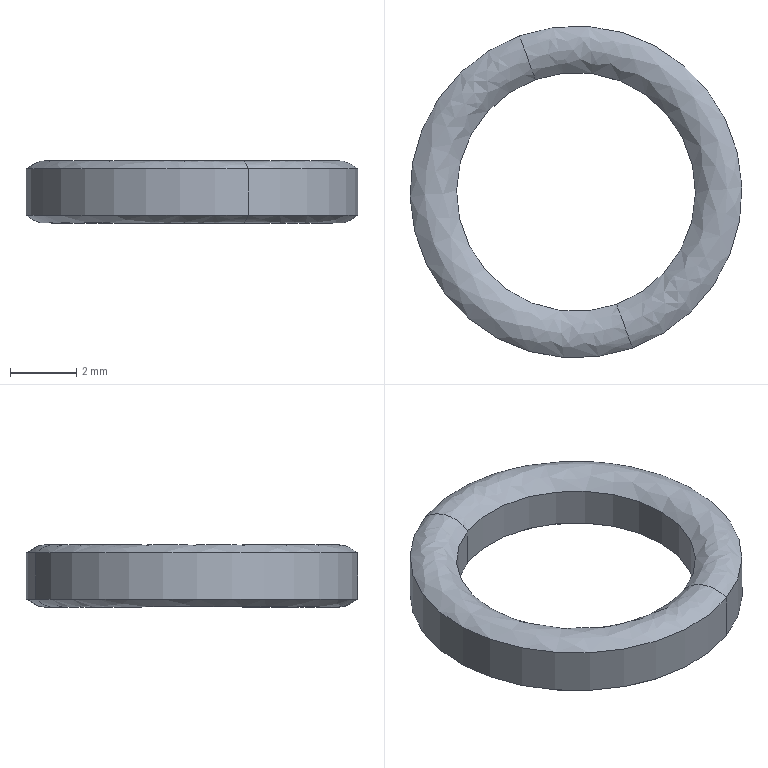Component | SolidWorks | NPB7-3 | 1 solid | 8 faces | box 10 x 10 x 1.9 mm | volume 65 mm3 | spline 4 | cylinder 4 | commonest cylinder face diameters 7.2 x2 10 x2
STEP:
#1=COLOUR_RGB('',0.7922,0.8196,0.9333);
#2=FILL_AREA_STYLE_COLOUR('',#1);
#3=FILL_AREA_STYLE('',(#2));
#4=SURFACE_STYLE_FILL_AREA(#3);
#5=SURFACE_SIDE_STYLE('',(#4));
#6=SURFACE_STYLE_USAGE(.BOTH.,#5);
#7=PRESENTATION_STYLE_ASSIGNMENT((#6));
#8=CARTESIAN_POINT('',(-0.06694,-1.587,0.3009));
#9=VERTEX_POINT('',#8);
#10=CARTESIAN_POINT('',(0.06694,-1.957,0.3009));
#11=VERTEX_POINT('',#10);
#12=CARTESIAN_POINT('',(0.,-1.772,0.3009));
#13=DIRECTION('',(-0.,-0.,1.));
#14=DIRECTION('',(-0.34,0.9404,0.));
#15=AXIS2_PLACEMENT_3D('',#12,#13,#14);
#16=CIRCLE('',#15,0.1969);
#17=EDGE_CURVE('',#9,#11,#16,.T.);
#18=ORIENTED_EDGE('',*,*,#17,.T.);
#19=CARTESIAN_POINT('',(0.04819,-1.905,0.2966));
#20=VERTEX_POINT('',#19);
#21=CARTESIAN_POINT('',(0.05823,-1.933,0.2736));
#22=DIRECTION('',(-0.9404,-0.34,-0.));
#23=DIRECTION('',(0.34,-0.9404,0.));
#24=AXIS2_PLACEMENT_3D('',#21,#22,#23);
#25=CIRCLE('',#24,0.0374);
#26=EDGE_CURVE('',#11,#20,#25,.T.);
#27=ORIENTED_EDGE('',*,*,#26,.T.);
#28=CARTESIAN_POINT('',(-0.04819,-1.638,0.2966));
#29=VERTEX_POINT('',#28);
#30=CARTESIAN_POINT('',(0.,-1.772,0.2966));
#31=DIRECTION('',(-0.,-0.,1.));
#32=DIRECTION('',(-0.34,0.9404,0.));
#33=AXIS2_PLACEMENT_3D('',#30,#31,#32);
#34=CIRCLE('',#33,0.1417);
#35=EDGE_CURVE('',#29,#20,#34,.T.);
#36=ORIENTED_EDGE('',*,*,#35,.F.);
#37=CARTESIAN_POINT('',(-0.05823,-1.611,0.2736));
#38=DIRECTION('',(0.9404,0.34,0.));
#39=DIRECTION('',(-0.34,0.9404,0.));
#40=AXIS2_PLACEMENT_3D('',#37,#38,#39);
#41=CIRCLE('',#40,0.0374);
#42=EDGE_CURVE('',#9,#29,#41,.T.);
#43=ORIENTED_EDGE('',*,*,#42,.F.);
#44=EDGE_LOOP('',(#18,#27,#36,#43));
#45=FACE_OUTER_BOUND('',#44,.T.);
#46=CARTESIAN_POINT('',(0.06694,-1.957,0.3009));
#47=CARTESIAN_POINT('',(-0.3033,-2.091,0.3009));
#48=CARTESIAN_POINT('',(-0.4372,-1.72,0.3009));
#49=CARTESIAN_POINT('',(-0.06694,-1.587,0.3009));
#50=CARTESIAN_POINT('',(0.06109,-1.941,0.317));
#51=CARTESIAN_POINT('',(-0.2768,-2.063,0.317));
#52=CARTESIAN_POINT('',(-0.399,-1.725,0.317));
#53=CARTESIAN_POINT('',(-0.06109,-1.603,0.317));
#54=CARTESIAN_POINT('',(0.05311,-1.919,0.3152));
#55=CARTESIAN_POINT('',(-0.2407,-2.025,0.3152));
#56=CARTESIAN_POINT('',(-0.3469,-1.731,0.3152));
#57=CARTESIAN_POINT('',(-0.05311,-1.625,0.3152));
#58=CARTESIAN_POINT('',(0.04819,-1.905,0.2966));
#59=CARTESIAN_POINT('',(-0.2184,-2.001,0.2966));
#60=CARTESIAN_POINT('',(-0.3148,-1.735,0.2966));
#61=CARTESIAN_POINT('',(-0.04819,-1.638,0.2966));
#62=(BOUNDED_SURFACE()B_SPLINE_SURFACE(3,3,((#46,#47,#48,#49),(#50,#51,#52,#53),(#54,#55,#56,#57),(#58,#59,#60,#61)),.UNSPECIFIED.,.F.,.F.,.T.)B_SPLINE_SURFACE_WITH_KNOTS((4,4),(4,4),(0.,1.),(0.,1.),.UNSPECIFIED.)GEOMETRIC_REPRESENTATION_ITEM()RATIONAL_B_SPLINE_SURFACE(((1.,0.3333,0.3333,1.),(0.7824,0.2608,0.2608,0.7824),(0.7824,0.2608,0.2608,0.7824),(1.,0.3333,0.3333,1.)))REPRESENTATION_ITEM('')SURFACE());
#63=ADVANCED_FACE('',(#45),#62,.T.);
#64=CARTESIAN_POINT('',(0.04819,-1.905,0.2507));
#65=VERTEX_POINT('',#64);
#66=CARTESIAN_POINT('',(-0.04819,-1.638,0.2507));
#67=VERTEX_POINT('',#66);
#68=CARTESIAN_POINT('',(0.,-1.772,0.2507));
#69=DIRECTION('',(0.,0.,-1.));
#70=DIRECTION('',(-0.34,0.9404,0.));
#71=AXIS2_PLACEMENT_3D('',#68,#69,#70);
#72=CIRCLE('',#71,0.1417);
#73=EDGE_CURVE('',#65,#67,#72,.T.);
#74=ORIENTED_EDGE('',*,*,#73,.F.);
#75=CARTESIAN_POINT('',(0.06694,-1.957,0.2463));
#76=VERTEX_POINT('',#75);
#77=CARTESIAN_POINT('',(0.05823,-1.933,0.2736));
#78=DIRECTION('',(-0.9404,-0.34,-0.));
#79=DIRECTION('',(0.34,-0.9404,0.));
#80=AXIS2_PLACEMENT_3D('',#77,#78,#79);
#81=CIRCLE('',#80,0.0374);
#82=EDGE_CURVE('',#65,#76,#81,.T.);
#83=ORIENTED_EDGE('',*,*,#82,.T.);
#84=CARTESIAN_POINT('',(-0.06694,-1.587,0.2463));
#85=VERTEX_POINT('',#84);
#86=CARTESIAN_POINT('',(0.,-1.772,0.2463));
#87=DIRECTION('',(0.,0.,-1.));
#88=DIRECTION('',(-0.34,0.9404,0.));
#89=AXIS2_PLACEMENT_3D('',#86,#87,#88);
#90=CIRCLE('',#89,0.1969);
#91=EDGE_CURVE('',#76,#85,#90,.T.);
#92=ORIENTED_EDGE('',*,*,#91,.T.);
#93=CARTESIAN_POINT('',(-0.05823,-1.611,0.2736));
#94=DIRECTION('',(0.9404,0.34,0.));
#95=DIRECTION('',(-0.34,0.9404,0.));
#96=AXIS2_PLACEMENT_3D('',#93,#94,#95);
#97=CIRCLE('',#96,0.0374);
#98=EDGE_CURVE('',#67,#85,#97,.T.);
#99=ORIENTED_EDGE('',*,*,#98,.F.);
#100=EDGE_LOOP('',(#74,#83,#92,#99));
#101=FACE_OUTER_BOUND('',#100,.T.);
#102=CARTESIAN_POINT('',(0.04819,-1.905,0.2507));
#103=CARTESIAN_POINT('',(-0.2184,-2.001,0.2507));
#104=CARTESIAN_POINT('',(-0.3148,-1.735,0.2507));
#105=CARTESIAN_POINT('',(-0.04819,-1.638,0.2507));
#106=CARTESIAN_POINT('',(0.05311,-1.919,0.2321));
#107=CARTESIAN_POINT('',(-0.2407,-2.025,0.2321));
#108=CARTESIAN_POINT('',(-0.3469,-1.731,0.2321));
#109=CARTESIAN_POINT('',(-0.05311,-1.625,0.2321));
#110=CARTESIAN_POINT('',(0.06109,-1.941,0.2302));
#111=CARTESIAN_POINT('',(-0.2768,-2.063,0.2302));
#112=CARTESIAN_POINT('',(-0.399,-1.725,0.2302));
#113=CARTESIAN_POINT('',(-0.06109,-1.603,0.2302));
#114=CARTESIAN_POINT('',(0.06694,-1.957,0.2463));
#115=CARTESIAN_POINT('',(-0.3033,-2.091,0.2463));
#116=CARTESIAN_POINT('',(-0.4372,-1.72,0.2463));
#117=CARTESIAN_POINT('',(-0.06694,-1.587,0.2463));
#118=(BOUNDED_SURFACE()B_SPLINE_SURFACE(3,3,((#102,#103,#104,#105),(#106,#107,#108,#109),(#110,#111,#112,#113),(#114,#115,#116,#117)),.UNSPECIFIED.,.F.,.F.,.T.)B_SPLINE_SURFACE_WITH_KNOTS((4,4),(4,4),(0.,1.),(0.,1.),.UNSPECIFIED.)GEOMETRIC_REPRESENTATION_ITEM()RATIONAL_B_SPLINE_SURFACE(((1.,0.3333,0.3333,1.),(0.7824,0.2608,0.2608,0.7824),(0.7824,0.2608,0.2608,0.7824),(1.,0.3333,0.3333,1.)))REPRESENTATION_ITEM('')SURFACE());
#119=ADVANCED_FACE('',(#101),#118,.T.);
#120=ORIENTED_EDGE('',*,*,#73,.T.);
#121=CARTESIAN_POINT('',(-0.04819,-1.638,0.1949));
#122=DIRECTION('',(-0.,-0.,1.));
#123=VECTOR('',#122,39.37);
#124=LINE('',#121,#123);
#125=EDGE_CURVE('',#67,#29,#124,.T.);
#126=ORIENTED_EDGE('',*,*,#125,.T.);
#127=ORIENTED_EDGE('',*,*,#35,.T.);
#128=CARTESIAN_POINT('',(0.04819,-1.905,0.1949));
#129=DIRECTION('',(-0.,-0.,1.));
#130=VECTOR('',#129,39.37);
#131=LINE('',#128,#130);
#132=EDGE_CURVE('',#65,#20,#131,.T.);
#133=ORIENTED_EDGE('',*,*,#132,.F.);
#134=EDGE_LOOP('',(#120,#126,#127,#133));
#135=FACE_OUTER_BOUND('',#134,.T.);
#136=CARTESIAN_POINT('',(0.,-1.772,0.1949));
#137=DIRECTION('',(-0.,-0.,1.));
#138=DIRECTION('',(0.34,-0.9404,0.));
#139=AXIS2_PLACEMENT_3D('',#136,#137,#138);
#140=CYLINDRICAL_SURFACE('',#139,0.1417);
#141=ADVANCED_FACE('',(#135),#140,.F.);
#142=CARTESIAN_POINT('',(0.,-1.772,0.2463));
#143=DIRECTION('',(0.,0.,-1.));
#144=DIRECTION('',(-0.34,0.9404,0.));
#145=AXIS2_PLACEMENT_3D('',#142,#143,#144);
#146=CIRCLE('',#145,0.1969);
#147=EDGE_CURVE('',#85,#76,#146,.T.);
#148=ORIENTED_EDGE('',*,*,#147,.F.);
#149=CARTESIAN_POINT('',(-0.06694,-1.587,0.1949));
#150=DIRECTION('',(-0.,-0.,1.));
#151=VECTOR('',#150,39.37);
#152=LINE('',#149,#151);
#153=EDGE_CURVE('',#85,#9,#152,.T.);
#154=ORIENTED_EDGE('',*,*,#153,.T.);
#155=CARTESIAN_POINT('',(0.,-1.772,0.3009));
#156=DIRECTION('',(-0.,-0.,1.));
#157=DIRECTION('',(-0.34,0.9404,0.));
#158=AXIS2_PLACEMENT_3D('',#155,#156,#157);
#159=CIRCLE('',#158,0.1969);
#160=EDGE_CURVE('',#11,#9,#159,.T.);
#161=ORIENTED_EDGE('',*,*,#160,.F.);
#162=CARTESIAN_POINT('',(0.06694,-1.957,0.1949));
#163=DIRECTION('',(-0.,-0.,1.));
#164=VECTOR('',#163,39.37);
#165=LINE('',#162,#164);
#166=EDGE_CURVE('',#76,#11,#165,.T.);
#167=ORIENTED_EDGE('',*,*,#166,.F.);
#168=EDGE_LOOP('',(#148,#154,#161,#167));
#169=FACE_OUTER_BOUND('',#168,.T.);
#170=CARTESIAN_POINT('',(0.,-1.772,0.1949));
#171=DIRECTION('',(-0.,-0.,1.));
#172=DIRECTION('',(0.34,-0.9404,0.));
#173=AXIS2_PLACEMENT_3D('',#170,#171,#172);
#174=CYLINDRICAL_SURFACE('',#173,0.1969);
#175=ADVANCED_FACE('',(#169),#174,.T.);
#176=ORIENTED_EDGE('',*,*,#82,.F.);
#177=CARTESIAN_POINT('',(0.,-1.772,0.2507));
#178=DIRECTION('',(0.,0.,-1.));
#179=DIRECTION('',(-0.34,0.9404,0.));
#180=AXIS2_PLACEMENT_3D('',#177,#178,#179);
#181=CIRCLE('',#180,0.1417);
#182=EDGE_CURVE('',#67,#65,#181,.T.);
#183=ORIENTED_EDGE('',*,*,#182,.F.);
#184=ORIENTED_EDGE('',*,*,#98,.T.);
#185=ORIENTED_EDGE('',*,*,#147,.T.);
#186=EDGE_LOOP('',(#176,#183,#184,#185));
#187=FACE_OUTER_BOUND('',#186,.T.);
#188=CARTESIAN_POINT('',(-0.04819,-1.638,0.2507));
#189=CARTESIAN_POINT('',(0.2184,-1.542,0.2507));
#190=CARTESIAN_POINT('',(0.3148,-1.809,0.2507));
#191=CARTESIAN_POINT('',(0.04819,-1.905,0.2507));
#192=CARTESIAN_POINT('',(-0.05311,-1.625,0.2321));
#193=CARTESIAN_POINT('',(0.2407,-1.519,0.2321));
#194=CARTESIAN_POINT('',(0.3469,-1.812,0.2321));
#195=CARTESIAN_POINT('',(0.05311,-1.919,0.2321));
#196=CARTESIAN_POINT('',(-0.06109,-1.603,0.2302));
#197=CARTESIAN_POINT('',(0.2768,-1.48,0.2302));
#198=CARTESIAN_POINT('',(0.399,-1.818,0.2302));
#199=CARTESIAN_POINT('',(0.06109,-1.941,0.2302));
#200=CARTESIAN_POINT('',(-0.06694,-1.587,0.2463));
#201=CARTESIAN_POINT('',(0.3033,-1.453,0.2463));
#202=CARTESIAN_POINT('',(0.4372,-1.823,0.2463));
#203=CARTESIAN_POINT('',(0.06694,-1.957,0.2463));
#204=(BOUNDED_SURFACE()B_SPLINE_SURFACE(3,3,((#188,#189,#190,#191),(#192,#193,#194,#195),(#196,#197,#198,#199),(#200,#201,#202,#203)),.UNSPECIFIED.,.F.,.F.,.F.)B_SPLINE_SURFACE_WITH_KNOTS((4,4),(4,4),(0.,1.),(0.,1.),.UNSPECIFIED.)GEOMETRIC_REPRESENTATION_ITEM()RATIONAL_B_SPLINE_SURFACE(((1.,0.3333,0.3333,1.),(0.7824,0.2608,0.2608,0.7824),(0.7824,0.2608,0.2608,0.7824),(1.,0.3333,0.3333,1.)))REPRESENTATION_ITEM('')SURFACE());
#205=ADVANCED_FACE('',(#187),#204,.T.);
#206=ORIENTED_EDGE('',*,*,#26,.F.);
#207=ORIENTED_EDGE('',*,*,#160,.T.);
#208=ORIENTED_EDGE('',*,*,#42,.T.);
#209=CARTESIAN_POINT('',(0.,-1.772,0.2966));
#210=DIRECTION('',(-0.,-0.,1.));
#211=DIRECTION('',(-0.34,0.9404,0.));
#212=AXIS2_PLACEMENT_3D('',#209,#210,#211);
#213=CIRCLE('',#212,0.1417);
#214=EDGE_CURVE('',#20,#29,#213,.T.);
#215=ORIENTED_EDGE('',*,*,#214,.F.);
#216=EDGE_LOOP('',(#206,#207,#208,#215));
#217=FACE_OUTER_BOUND('',#216,.T.);
#218=CARTESIAN_POINT('',(-0.06694,-1.587,0.3009));
#219=CARTESIAN_POINT('',(0.3033,-1.453,0.3009));
#220=CARTESIAN_POINT('',(0.4372,-1.823,0.3009));
#221=CARTESIAN_POINT('',(0.06694,-1.957,0.3009));
#222=CARTESIAN_POINT('',(-0.06109,-1.603,0.317));
#223=CARTESIAN_POINT('',(0.2768,-1.48,0.317));
#224=CARTESIAN_POINT('',(0.399,-1.818,0.317));
#225=CARTESIAN_POINT('',(0.06109,-1.941,0.317));
#226=CARTESIAN_POINT('',(-0.05311,-1.625,0.3152));
#227=CARTESIAN_POINT('',(0.2407,-1.519,0.3152));
#228=CARTESIAN_POINT('',(0.3469,-1.812,0.3152));
#229=CARTESIAN_POINT('',(0.05311,-1.919,0.3152));
#230=CARTESIAN_POINT('',(-0.04819,-1.638,0.2966));
#231=CARTESIAN_POINT('',(0.2184,-1.542,0.2966));
#232=CARTESIAN_POINT('',(0.3148,-1.809,0.2966));
#233=CARTESIAN_POINT('',(0.04819,-1.905,0.2966));
#234=(BOUNDED_SURFACE()B_SPLINE_SURFACE(3,3,((#218,#219,#220,#221),(#222,#223,#224,#225),(#226,#227,#228,#229),(#230,#231,#232,#233)),.UNSPECIFIED.,.F.,.F.,.T.)B_SPLINE_SURFACE_WITH_KNOTS((4,4),(4,4),(0.,1.),(0.,1.),.UNSPECIFIED.)GEOMETRIC_REPRESENTATION_ITEM()RATIONAL_B_SPLINE_SURFACE(((1.,0.3333,0.3333,1.),(0.7824,0.2608,0.2608,0.7824),(0.7824,0.2608,0.2608,0.7824),(1.,0.3333,0.3333,1.)))REPRESENTATION_ITEM('')SURFACE());
#235=ADVANCED_FACE('',(#217),#234,.T.);
#236=ORIENTED_EDGE('',*,*,#153,.F.);
#237=ORIENTED_EDGE('',*,*,#91,.F.);
#238=ORIENTED_EDGE('',*,*,#166,.T.);
#239=ORIENTED_EDGE('',*,*,#17,.F.);
#240=EDGE_LOOP('',(#236,#237,#238,#239));
#241=FACE_OUTER_BOUND('',#240,.T.);
#242=CARTESIAN_POINT('',(0.,-1.772,0.1949));
#243=DIRECTION('',(-0.,-0.,1.));
#244=DIRECTION('',(0.34,-0.9404,0.));
#245=AXIS2_PLACEMENT_3D('',#242,#243,#244);
#246=CYLINDRICAL_SURFACE('',#245,0.1969);
#247=ADVANCED_FACE('',(#241),#246,.T.);
#248=ORIENTED_EDGE('',*,*,#125,.F.);
#249=ORIENTED_EDGE('',*,*,#182,.T.);
#250=ORIENTED_EDGE('',*,*,#132,.T.);
#251=ORIENTED_EDGE('',*,*,#214,.T.);
#252=EDGE_LOOP('',(#248,#249,#250,#251));
#253=FACE_OUTER_BOUND('',#252,.T.);
#254=CARTESIAN_POINT('',(0.,-1.772,0.1949));
#255=DIRECTION('',(-0.,-0.,1.));
#256=DIRECTION('',(0.34,-0.9404,0.));
#257=AXIS2_PLACEMENT_3D('',#254,#255,#256);
#258=CYLINDRICAL_SURFACE('',#257,0.1417);
#259=ADVANCED_FACE('',(#253),#258,.F.);
#260=CLOSED_SHELL('',(#63,#119,#141,#175,#205,#235,#247,#259));
#261=MANIFOLD_SOLID_BREP('',#260);
#262=STYLED_ITEM('',(#7),#261);
#263=PRESENTATION_LAYER_ASSIGNMENT('','',(#262));
#264=CARTESIAN_POINT('',(0.,0.,0.));
#265=DIRECTION('',(0.,0.,1.));
#266=DIRECTION('',(1.,0.,0.));
#267=AXIS2_PLACEMENT_3D('',#264,#265,#266);
#268=(LENGTH_UNIT()NAMED_UNIT(*)SI_UNIT($,.METRE.));
#269=LENGTH_MEASURE_WITH_UNIT(LENGTH_MEASURE(0.0254),#268);
#270=DIMENSIONAL_EXPONENTS(1.,0.,0.,0.,0.,0.,0.);
#271=(CONVERSION_BASED_UNIT('',#269)LENGTH_UNIT()NAMED_UNIT(#270));
#272=UNCERTAINTY_MEASURE_WITH_UNIT(LENGTH_MEASURE(0.00001),#271,'','');
#273=(NAMED_UNIT(*)PLANE_ANGLE_UNIT()SI_UNIT($,.RADIAN.));
#274=(NAMED_UNIT(*)SI_UNIT($,.STERADIAN.)SOLID_ANGLE_UNIT());
#275=(GEOMETRIC_REPRESENTATION_CONTEXT(3)GLOBAL_UNCERTAINTY_ASSIGNED_CONTEXT((#272))GLOBAL_UNIT_ASSIGNED_CONTEXT((#271,#273,#274))REPRESENTATION_CONTEXT('',''));
#276=ADVANCED_BREP_SHAPE_REPRESENTATION('',(#261,#267),#275);
#277=(LENGTH_UNIT()NAMED_UNIT(*)SI_UNIT($,.METRE.));
#278=LENGTH_MEASURE_WITH_UNIT(LENGTH_MEASURE(0.0254),#277);
#279=DIMENSIONAL_EXPONENTS(1.,0.,0.,0.,0.,0.,0.);
#280=(CONVERSION_BASED_UNIT('',#278)LENGTH_UNIT()NAMED_UNIT(#279));
#281=UNCERTAINTY_MEASURE_WITH_UNIT(LENGTH_MEASURE(0.00001),#280,'','');
#282=(NAMED_UNIT(*)PLANE_ANGLE_UNIT()SI_UNIT($,.RADIAN.));
#283=(NAMED_UNIT(*)SI_UNIT($,.STERADIAN.)SOLID_ANGLE_UNIT());
#284=(GEOMETRIC_REPRESENTATION_CONTEXT(3)GLOBAL_UNCERTAINTY_ASSIGNED_CONTEXT((#281))GLOBAL_UNIT_ASSIGNED_CONTEXT((#280,#282,#283))REPRESENTATION_CONTEXT('',''));
#285=MECHANICAL_DESIGN_GEOMETRIC_PRESENTATION_REPRESENTATION('',(#262),#284);